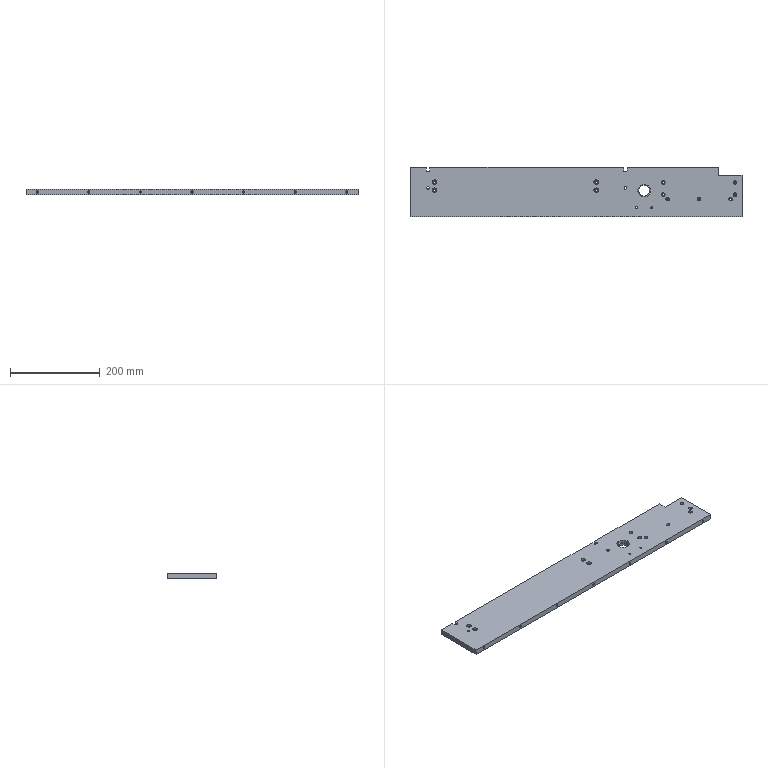Component | SolidWorks | LD101-02--Q1051-Q1-2-1 | 1 solid | 122 faces | box 740 x 110 x 12 mm | volume 947716 mm3 | cylinder 78 | plane 26 | cone 18 | commonest cylinder face diameters 5 x18 8 x14 4.5 x14 10 x8 5.5 x8 4.2 x4 6 x4 8.2 x4 | material AL6061
build123d program:
from build123d import *

# Parameters (mm, degrees)
SKETCH1_W                                          = 740
SKETCH1_H                                          = 110
BOSS_EXTRUDE1_DEPTH                                = 6
CUT_EXTRUDE1_DEPTH                                 = 375.258
M5_TAPPED_HOLE2_D                                  = 6
SKETCH11_R                                         = 14
CUT_EXTRUDE2_DEPTH                                 = 7
SKETCH12_R                                         = 12
CUT_EXTRUDE3_DEPTH                                 = 375.131
SKETCH13_W                                         = 52
SKETCH13_H                                         = 18
CUT_EXTRUDE4_DEPTH                                 = 375.258
HOLE_SIZE_FOR_HEX_SOCKET_HEAD_CAP_SCRE_D           = 4.5
HOLE_SIZE_FOR_HEX_SOCKET_HEAD_CAP_SCRE_CBORE_D     = 8
HOLE_SIZE_FOR_HEX_SOCKET_HEAD_CAP_SCRE_CBORE_DEPTH = 4.6
M6_TAPPED_HOLE1_D                                  = 5
M6_TAPPED_HOLE1_DEPTH                              = 20
M6_TAPPED_HOLE1_TIP                                = 1.502
M6_TAPPED_HOLE2_D                                  = 5
M6_TAPPED_HOLE2_DEPTH                              = 20
M6_TAPPED_HOLE2_TIP                                = 1.502
HOLE_SIZE_FOR_HEX_SOCKET_HEAD_CAP_2_D              = 5.5
HOLE_SIZE_FOR_HEX_SOCKET_HEAD_CAP_2_CBORE_D        = 10
HOLE_SIZE_FOR_HEX_SOCKET_HEAD_CAP_2_CBORE_DEPTH    = 5.7
M5_TAPPED_HOLE3_D                                  = 4.2


with BuildPart() as part:
    # Sketch1 → Boss-Extrude1 (new, symmetric)
    with BuildSketch(Plane(origin=(0, 0, 0), x_dir=(1, 0, 0), z_dir=(0, 1, 0))):
        Rectangle(SKETCH1_W, SKETCH1_H)
    extrude(amount=BOSS_EXTRUDE1_DEPTH, both=True)

    # Sketch2 → Cut-Extrude1 (cut, through all)
    with BuildSketch(Plane.XZ.offset(6)):
        with BuildLine():
            Line((-325.9, 55), (-325.9, 49))
            ThreePointArc((-325.9, 49), (-330, 44.9), (-334.1, 49))
            Line((-334.1, 49), (-334.1, 55))
            ThreePointArc((-334.1, 55), (-330, 59.1), (-325.9, 55))
        make_face()
        with BuildLine():
            Line((105.9, 55), (105.9, 49))
            ThreePointArc((105.9, 49), (110, 44.9), (114.1, 49))
            Line((114.1, 49), (114.1, 55))
            ThreePointArc((114.1, 55), (110, 59.1), (105.9, 55))
        make_face()
    extrude(amount=-CUT_EXTRUDE1_DEPTH, mode=Mode.SUBTRACT)

    # M5 Tapped Hole2 (through all)
    with Locations(Plane(origin=(0, -6, 0), x_dir=(-1, 0, 0), z_dir=(0, -1, 0))):
        with Locations((-110, -9), (330, -9)):
            Hole(M5_TAPPED_HOLE2_D / 2)

    # Sketch11 → Cut-Extrude2 (cut)
    with BuildSketch(Plane.XZ.offset(6)):
        with Locations(Location((152, 3, 0), (0, 0, 270))):
            Circle(SKETCH11_R)
    extrude(amount=-CUT_EXTRUDE2_DEPTH, mode=Mode.SUBTRACT)

    # Sketch12 → Cut-Extrude3 (cut, through all)
    with BuildSketch(Plane.XZ.offset(-1)):
        with Locations(Location((152, 3, 0), (0, 0, 270))):
            Circle(SKETCH12_R)
    extrude(amount=-CUT_EXTRUDE3_DEPTH, mode=Mode.SUBTRACT)

    # Sketch13 → Cut-Extrude4 (cut, through all)
    with BuildSketch(Plane.XZ.offset(6)):
        with Locations((344, 46)):
            Rectangle(SKETCH13_W, SKETCH13_H)
    extrude(amount=-CUT_EXTRUDE4_DEPTH, mode=Mode.SUBTRACT)

    # Hole Size _for_ Hex Socket Head Cap Scre (through all)
    with Locations(Plane(origin=(0, -6, 0), x_dir=(-1, 0, 0), z_dir=(0, -1, 0))):
        with Locations((-344.5, 16), (-274.5, 16), (-354.5, 6), (-354.5, -21), (-194.5, -21), (-194.5, 6), (-204.5, 16)):
            CounterBoreHole(HOLE_SIZE_FOR_HEX_SOCKET_HEAD_CAP_SCRE_D / 2, HOLE_SIZE_FOR_HEX_SOCKET_HEAD_CAP_SCRE_CBORE_D / 2, HOLE_SIZE_FOR_HEX_SOCKET_HEAD_CAP_SCRE_CBORE_DEPTH)

    # M6 Tapped Hole1
    with Locations(Plane.XY.offset(37)):
        with Locations((362, 0), (347, 0)):
            Hole(M6_TAPPED_HOLE1_D / 2, depth=M6_TAPPED_HOLE1_DEPTH)
            with Locations((0, 0, -(M6_TAPPED_HOLE1_DEPTH + M6_TAPPED_HOLE1_TIP / 2))):  # 118° drill point
                Cone(0, M6_TAPPED_HOLE1_D / 2, M6_TAPPED_HOLE1_TIP, mode=Mode.SUBTRACT)

    # M6 Tapped Hole2
    with Locations(Plane(origin=(0, 0, -55), x_dir=(-1, 0, 0), z_dir=(0, 0, -1))):
        with Locations((0, 0), (-115, 0), (-230, 0), (230, 0), (115, 0), (-345, 0), (345, 0)):
            Hole(M6_TAPPED_HOLE2_D / 2, depth=M6_TAPPED_HOLE2_DEPTH)
            with Locations((0, 0, -(M6_TAPPED_HOLE2_DEPTH + M6_TAPPED_HOLE2_TIP / 2))):  # 118° drill point
                Cone(0, M6_TAPPED_HOLE2_D / 2, M6_TAPPED_HOLE2_TIP, mode=Mode.SUBTRACT)

    # Hole Size _for_ Hex Socket Head Cap  2 (through all)
    with Locations(Plane(origin=(0, -6, 0), x_dir=(-1, 0, 0), z_dir=(0, -1, 0))):
        with Locations((315, -22), (315, -4), (-45, -22), (-45, -4)):
            CounterBoreHole(HOLE_SIZE_FOR_HEX_SOCKET_HEAD_CAP_2_D / 2, HOLE_SIZE_FOR_HEX_SOCKET_HEAD_CAP_2_CBORE_D / 2, HOLE_SIZE_FOR_HEX_SOCKET_HEAD_CAP_2_CBORE_DEPTH)

    # M5 Tapped Hole3 (through all)
    with Locations(Plane(origin=(0, -6, 0), x_dir=(-1, 0, 0), z_dir=(0, -1, 0))):
        with Locations((-135, 35), (-169, 35)):
            Hole(M5_TAPPED_HOLE3_D / 2)


solid = part.part

# Placed as in the assembly
solid = solid.moved(Location((-30.29, -184.897, 287.257), (-90, 0, 0)))